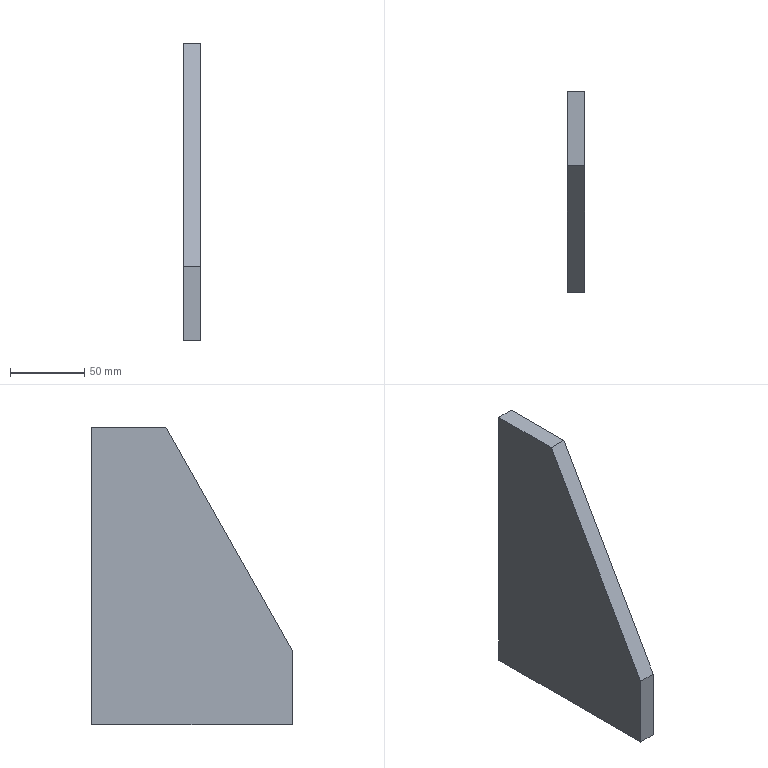Component | SolidWorks | FlangeRib1-2 | 1 solid | 7 faces | box 12 x 135 x 200 mm | volume 247500 mm3 | plane 7 | material Plain Carbon Steel
STEP:
#1=CARTESIAN_POINT('',(39.157,36.667,61.46));
#2=VERTEX_POINT('',#1);
#3=CARTESIAN_POINT('',(39.157,36.667,63.429));
#4=VERTEX_POINT('',#3);
#5=CARTESIAN_POINT('',(39.157,36.667,63.429));
#6=DIRECTION('',(-0.,0.,1.));
#7=VECTOR('',#6,39.37);
#8=LINE('',#5,#7);
#9=EDGE_CURVE('',#2,#4,#8,.T.);
#10=ORIENTED_EDGE('',*,*,#9,.F.);
#11=CARTESIAN_POINT('',(39.629,36.667,61.46));
#12=VERTEX_POINT('',#11);
#13=CARTESIAN_POINT('',(39.629,36.667,61.46));
#14=DIRECTION('',(-1.,0.,-0.));
#15=VECTOR('',#14,39.37);
#16=LINE('',#13,#15);
#17=EDGE_CURVE('',#12,#2,#16,.T.);
#18=ORIENTED_EDGE('',*,*,#17,.F.);
#19=CARTESIAN_POINT('',(39.629,36.667,63.429));
#20=VERTEX_POINT('',#19);
#21=CARTESIAN_POINT('',(39.629,36.667,63.429));
#22=DIRECTION('',(-0.,0.,1.));
#23=VECTOR('',#22,39.37);
#24=LINE('',#21,#23);
#25=EDGE_CURVE('',#12,#20,#24,.T.);
#26=ORIENTED_EDGE('',*,*,#25,.T.);
#27=CARTESIAN_POINT('',(39.629,36.667,63.429));
#28=DIRECTION('',(-1.,0.,-0.));
#29=VECTOR('',#28,39.37);
#30=LINE('',#27,#29);
#31=EDGE_CURVE('',#20,#4,#30,.T.);
#32=ORIENTED_EDGE('',*,*,#31,.T.);
#33=EDGE_LOOP('',(#10,#18,#26,#32));
#34=FACE_OUTER_BOUND('',#33,.T.);
#35=CARTESIAN_POINT('',(39.629,36.667,63.429));
#36=DIRECTION('',(-0.,-1.,0.));
#37=DIRECTION('',(-1.,0.,-0.));
#38=AXIS2_PLACEMENT_3D('',#35,#36,#37);
#39=PLANE('',#38);
#40=ADVANCED_FACE('',(#34),#39,.T.);
#41=CARTESIAN_POINT('',(39.157,41.982,61.46));
#42=VERTEX_POINT('',#41);
#43=CARTESIAN_POINT('',(39.157,36.667,61.46));
#44=DIRECTION('',(-0.,-1.,0.));
#45=VECTOR('',#44,39.37);
#46=LINE('',#43,#45);
#47=EDGE_CURVE('',#42,#2,#46,.T.);
#48=ORIENTED_EDGE('',*,*,#47,.F.);
#49=CARTESIAN_POINT('',(39.629,41.982,61.46));
#50=VERTEX_POINT('',#49);
#51=CARTESIAN_POINT('',(39.629,41.982,61.46));
#52=DIRECTION('',(-1.,0.,-0.));
#53=VECTOR('',#52,39.37);
#54=LINE('',#51,#53);
#55=EDGE_CURVE('',#50,#42,#54,.T.);
#56=ORIENTED_EDGE('',*,*,#55,.F.);
#57=CARTESIAN_POINT('',(39.629,36.667,61.46));
#58=DIRECTION('',(-0.,-1.,0.));
#59=VECTOR('',#58,39.37);
#60=LINE('',#57,#59);
#61=EDGE_CURVE('',#50,#12,#60,.T.);
#62=ORIENTED_EDGE('',*,*,#61,.T.);
#63=ORIENTED_EDGE('',*,*,#17,.T.);
#64=EDGE_LOOP('',(#48,#56,#62,#63));
#65=FACE_OUTER_BOUND('',#64,.T.);
#66=CARTESIAN_POINT('',(39.629,36.667,61.46));
#67=DIRECTION('',(0.,-0.,-1.));
#68=DIRECTION('',(-0.,-1.,0.));
#69=AXIS2_PLACEMENT_3D('',#66,#67,#68);
#70=PLANE('',#69);
#71=ADVANCED_FACE('',(#65),#70,.T.);
#72=CARTESIAN_POINT('',(39.157,41.982,69.334));
#73=VERTEX_POINT('',#72);
#74=CARTESIAN_POINT('',(39.157,41.982,61.46));
#75=DIRECTION('',(0.,-0.,-1.));
#76=VECTOR('',#75,39.37);
#77=LINE('',#74,#76);
#78=EDGE_CURVE('',#73,#42,#77,.T.);
#79=ORIENTED_EDGE('',*,*,#78,.F.);
#80=CARTESIAN_POINT('',(39.629,41.982,69.334));
#81=VERTEX_POINT('',#80);
#82=CARTESIAN_POINT('',(39.629,41.982,69.334));
#83=DIRECTION('',(-1.,0.,-0.));
#84=VECTOR('',#83,39.37);
#85=LINE('',#82,#84);
#86=EDGE_CURVE('',#81,#73,#85,.T.);
#87=ORIENTED_EDGE('',*,*,#86,.F.);
#88=CARTESIAN_POINT('',(39.629,41.982,61.46));
#89=DIRECTION('',(0.,-0.,-1.));
#90=VECTOR('',#89,39.37);
#91=LINE('',#88,#90);
#92=EDGE_CURVE('',#81,#50,#91,.T.);
#93=ORIENTED_EDGE('',*,*,#92,.T.);
#94=ORIENTED_EDGE('',*,*,#55,.T.);
#95=EDGE_LOOP('',(#79,#87,#93,#94));
#96=FACE_OUTER_BOUND('',#95,.T.);
#97=CARTESIAN_POINT('',(39.629,41.982,61.46));
#98=DIRECTION('',(0.,1.,-0.));
#99=DIRECTION('',(0.,-0.,-1.));
#100=AXIS2_PLACEMENT_3D('',#97,#98,#99);
#101=PLANE('',#100);
#102=ADVANCED_FACE('',(#96),#101,.T.);
#103=CARTESIAN_POINT('',(39.157,40.014,69.334));
#104=VERTEX_POINT('',#103);
#105=CARTESIAN_POINT('',(39.157,41.982,69.334));
#106=DIRECTION('',(0.,1.,-0.));
#107=VECTOR('',#106,39.37);
#108=LINE('',#105,#107);
#109=EDGE_CURVE('',#104,#73,#108,.T.);
#110=ORIENTED_EDGE('',*,*,#109,.F.);
#111=CARTESIAN_POINT('',(39.629,40.014,69.334));
#112=VERTEX_POINT('',#111);
#113=CARTESIAN_POINT('',(39.629,40.014,69.334));
#114=DIRECTION('',(-1.,0.,-0.));
#115=VECTOR('',#114,39.37);
#116=LINE('',#113,#115);
#117=EDGE_CURVE('',#112,#104,#116,.T.);
#118=ORIENTED_EDGE('',*,*,#117,.F.);
#119=CARTESIAN_POINT('',(39.629,41.982,69.334));
#120=DIRECTION('',(0.,1.,-0.));
#121=VECTOR('',#120,39.37);
#122=LINE('',#119,#121);
#123=EDGE_CURVE('',#112,#81,#122,.T.);
#124=ORIENTED_EDGE('',*,*,#123,.T.);
#125=ORIENTED_EDGE('',*,*,#86,.T.);
#126=EDGE_LOOP('',(#110,#118,#124,#125));
#127=FACE_OUTER_BOUND('',#126,.T.);
#128=CARTESIAN_POINT('',(39.629,41.982,69.334));
#129=DIRECTION('',(-0.,0.,1.));
#130=DIRECTION('',(0.,1.,-0.));
#131=AXIS2_PLACEMENT_3D('',#128,#129,#130);
#132=PLANE('',#131);
#133=ADVANCED_FACE('',(#127),#132,.T.);
#134=CARTESIAN_POINT('',(39.157,40.014,69.334));
#135=DIRECTION('',(-0.,0.493,0.87));
#136=VECTOR('',#135,39.37);
#137=LINE('',#134,#136);
#138=EDGE_CURVE('',#4,#104,#137,.T.);
#139=ORIENTED_EDGE('',*,*,#138,.F.);
#140=ORIENTED_EDGE('',*,*,#31,.F.);
#141=CARTESIAN_POINT('',(39.629,40.014,69.334));
#142=DIRECTION('',(-0.,0.493,0.87));
#143=VECTOR('',#142,39.37);
#144=LINE('',#141,#143);
#145=EDGE_CURVE('',#20,#112,#144,.T.);
#146=ORIENTED_EDGE('',*,*,#145,.T.);
#147=ORIENTED_EDGE('',*,*,#117,.T.);
#148=EDGE_LOOP('',(#139,#140,#146,#147));
#149=FACE_OUTER_BOUND('',#148,.T.);
#150=CARTESIAN_POINT('',(39.629,40.014,69.334));
#151=DIRECTION('',(-0.,-0.87,0.493));
#152=DIRECTION('',(-0.,0.493,0.87));
#153=AXIS2_PLACEMENT_3D('',#150,#151,#152);
#154=PLANE('',#153);
#155=ADVANCED_FACE('',(#149),#154,.T.);
#156=ORIENTED_EDGE('',*,*,#25,.F.);
#157=ORIENTED_EDGE('',*,*,#61,.F.);
#158=ORIENTED_EDGE('',*,*,#92,.F.);
#159=ORIENTED_EDGE('',*,*,#123,.F.);
#160=ORIENTED_EDGE('',*,*,#145,.F.);
#161=EDGE_LOOP('',(#156,#157,#158,#159,#160));
#162=FACE_OUTER_BOUND('',#161,.T.);
#163=CARTESIAN_POINT('',(39.629,36.667,61.46));
#164=DIRECTION('',(1.,0.,0.));
#165=DIRECTION('',(-0.,-1.,0.));
#166=AXIS2_PLACEMENT_3D('',#163,#164,#165);
#167=PLANE('',#166);
#168=ADVANCED_FACE('',(#162),#167,.T.);
#169=ORIENTED_EDGE('',*,*,#9,.T.);
#170=ORIENTED_EDGE('',*,*,#138,.T.);
#171=ORIENTED_EDGE('',*,*,#109,.T.);
#172=ORIENTED_EDGE('',*,*,#78,.T.);
#173=ORIENTED_EDGE('',*,*,#47,.T.);
#174=EDGE_LOOP('',(#169,#170,#171,#172,#173));
#175=FACE_OUTER_BOUND('',#174,.T.);
#176=CARTESIAN_POINT('',(39.157,36.667,61.46));
#177=DIRECTION('',(1.,0.,0.));
#178=DIRECTION('',(-0.,-1.,0.));
#179=AXIS2_PLACEMENT_3D('',#176,#177,#178);
#180=PLANE('',#179);
#181=ADVANCED_FACE('',(#175),#180,.F.);
#182=CLOSED_SHELL('',(#40,#71,#102,#133,#155,#168,#181));
#183=MANIFOLD_SOLID_BREP('',#182);
#184=CARTESIAN_POINT('',(0.,0.,0.));
#185=DIRECTION('',(0.,0.,1.));
#186=DIRECTION('',(1.,0.,0.));
#187=AXIS2_PLACEMENT_3D('',#184,#185,#186);
#188=(LENGTH_UNIT()NAMED_UNIT(*)SI_UNIT($,.METRE.));
#189=LENGTH_MEASURE_WITH_UNIT(LENGTH_MEASURE(0.0254),#188);
#190=DIMENSIONAL_EXPONENTS(1.,0.,0.,0.,0.,0.,0.);
#191=(CONVERSION_BASED_UNIT('',#189)LENGTH_UNIT()NAMED_UNIT(#190));
#192=UNCERTAINTY_MEASURE_WITH_UNIT(LENGTH_MEASURE(0.00001),#191,'','');
#193=(NAMED_UNIT(*)PLANE_ANGLE_UNIT()SI_UNIT($,.RADIAN.));
#194=(NAMED_UNIT(*)SI_UNIT($,.STERADIAN.)SOLID_ANGLE_UNIT());
#195=(GEOMETRIC_REPRESENTATION_CONTEXT(3)GLOBAL_UNCERTAINTY_ASSIGNED_CONTEXT((#192))GLOBAL_UNIT_ASSIGNED_CONTEXT((#191,#193,#194))REPRESENTATION_CONTEXT('',''));
#196=ADVANCED_BREP_SHAPE_REPRESENTATION('',(#183,#187),#195);
#197=COLOUR_RGB('',0.7922,0.8196,0.9333);
#198=FILL_AREA_STYLE_COLOUR('',#197);
#199=FILL_AREA_STYLE('',(#198));
#200=SURFACE_STYLE_FILL_AREA(#199);
#201=SURFACE_SIDE_STYLE('',(#200));
#202=SURFACE_STYLE_USAGE(.BOTH.,#201);
#203=PRESENTATION_STYLE_ASSIGNMENT((#202));
#204=STYLED_ITEM('',(#203),#183);
#205=PRESENTATION_LAYER_ASSIGNMENT('','',(#204));
#206=(LENGTH_UNIT()NAMED_UNIT(*)SI_UNIT($,.METRE.));
#207=LENGTH_MEASURE_WITH_UNIT(LENGTH_MEASURE(0.0254),#206);
#208=DIMENSIONAL_EXPONENTS(1.,0.,0.,0.,0.,0.,0.);
#209=(CONVERSION_BASED_UNIT('',#207)LENGTH_UNIT()NAMED_UNIT(#208));
#210=UNCERTAINTY_MEASURE_WITH_UNIT(LENGTH_MEASURE(0.00001),#209,'','');
#211=(NAMED_UNIT(*)PLANE_ANGLE_UNIT()SI_UNIT($,.RADIAN.));
#212=(NAMED_UNIT(*)SI_UNIT($,.STERADIAN.)SOLID_ANGLE_UNIT());
#213=(GEOMETRIC_REPRESENTATION_CONTEXT(3)GLOBAL_UNCERTAINTY_ASSIGNED_CONTEXT((#210))GLOBAL_UNIT_ASSIGNED_CONTEXT((#209,#211,#212))REPRESENTATION_CONTEXT('',''));
#214=MECHANICAL_DESIGN_GEOMETRIC_PRESENTATION_REPRESENTATION('',(#204),#213);